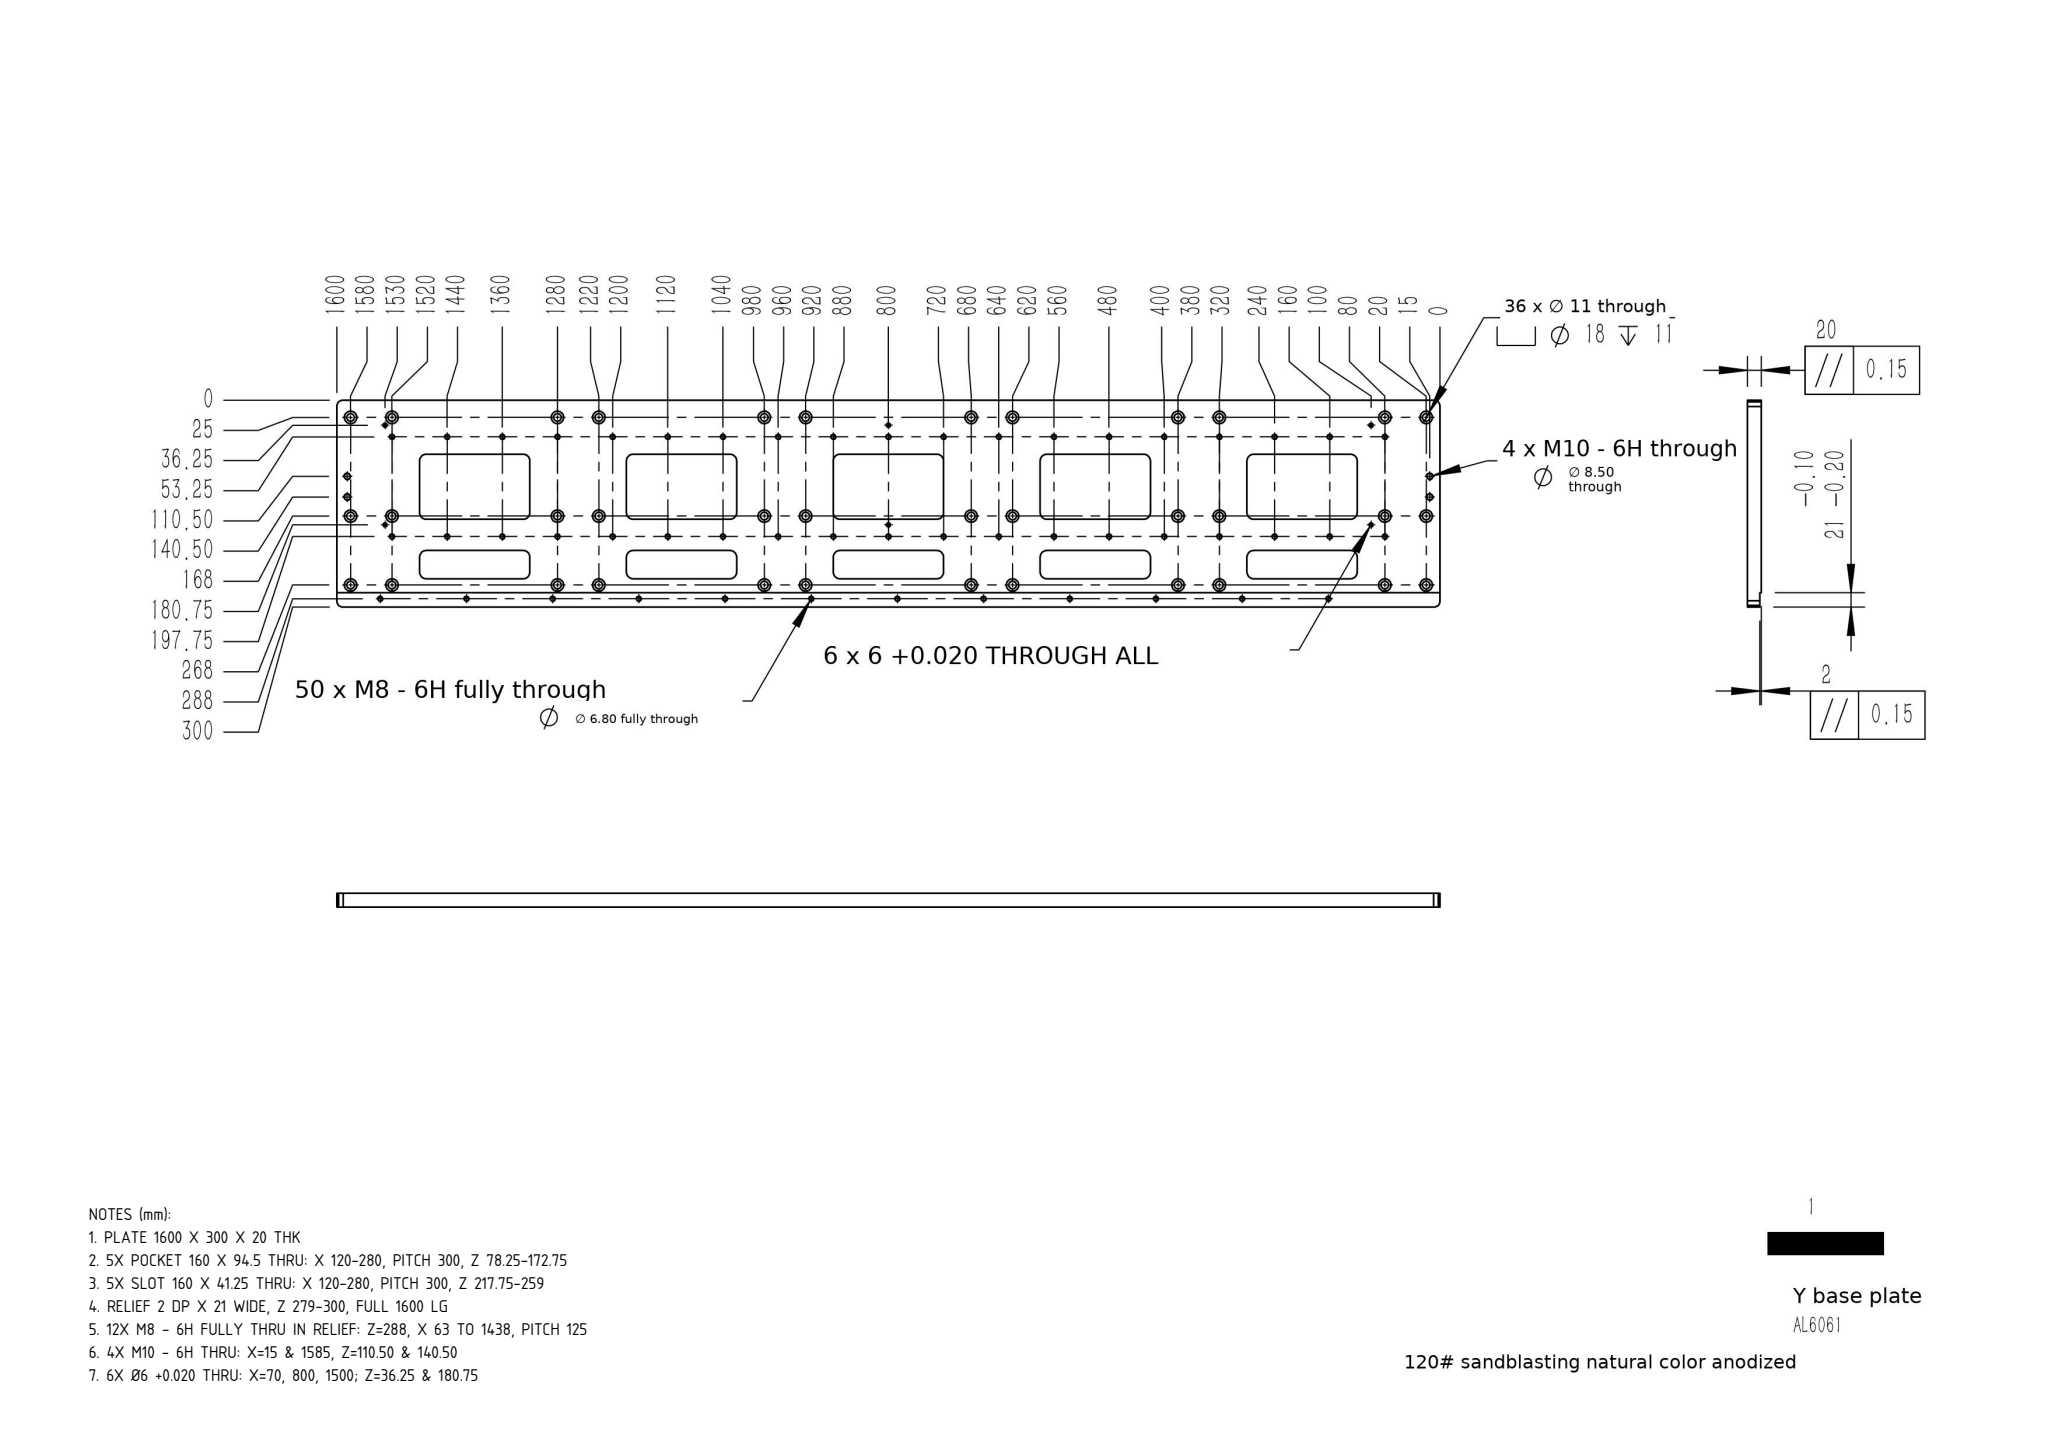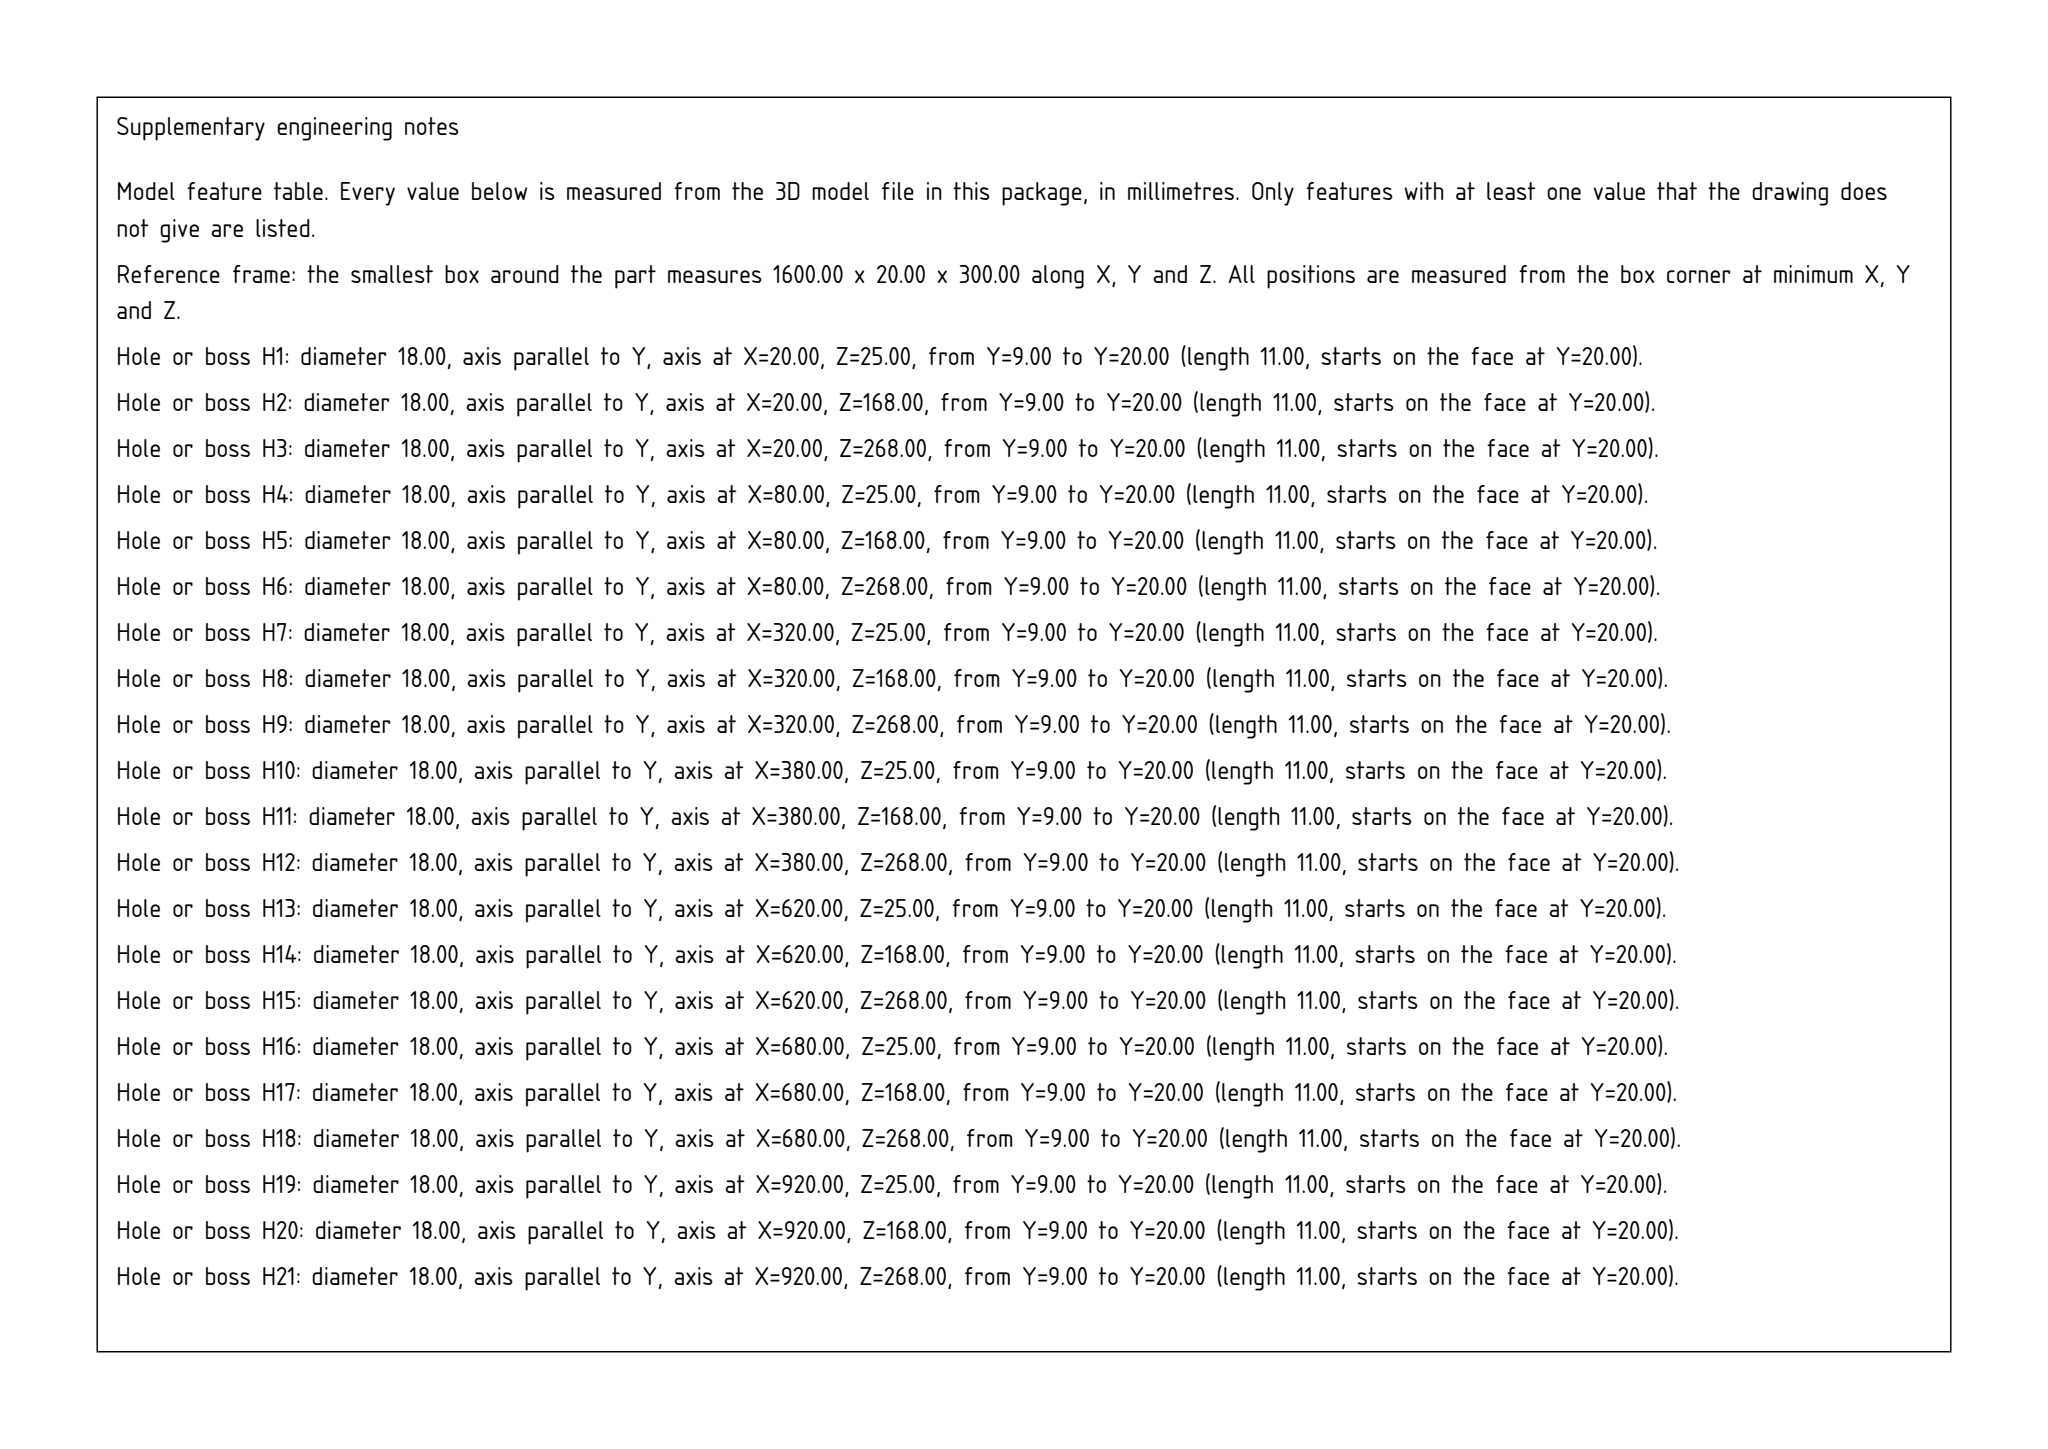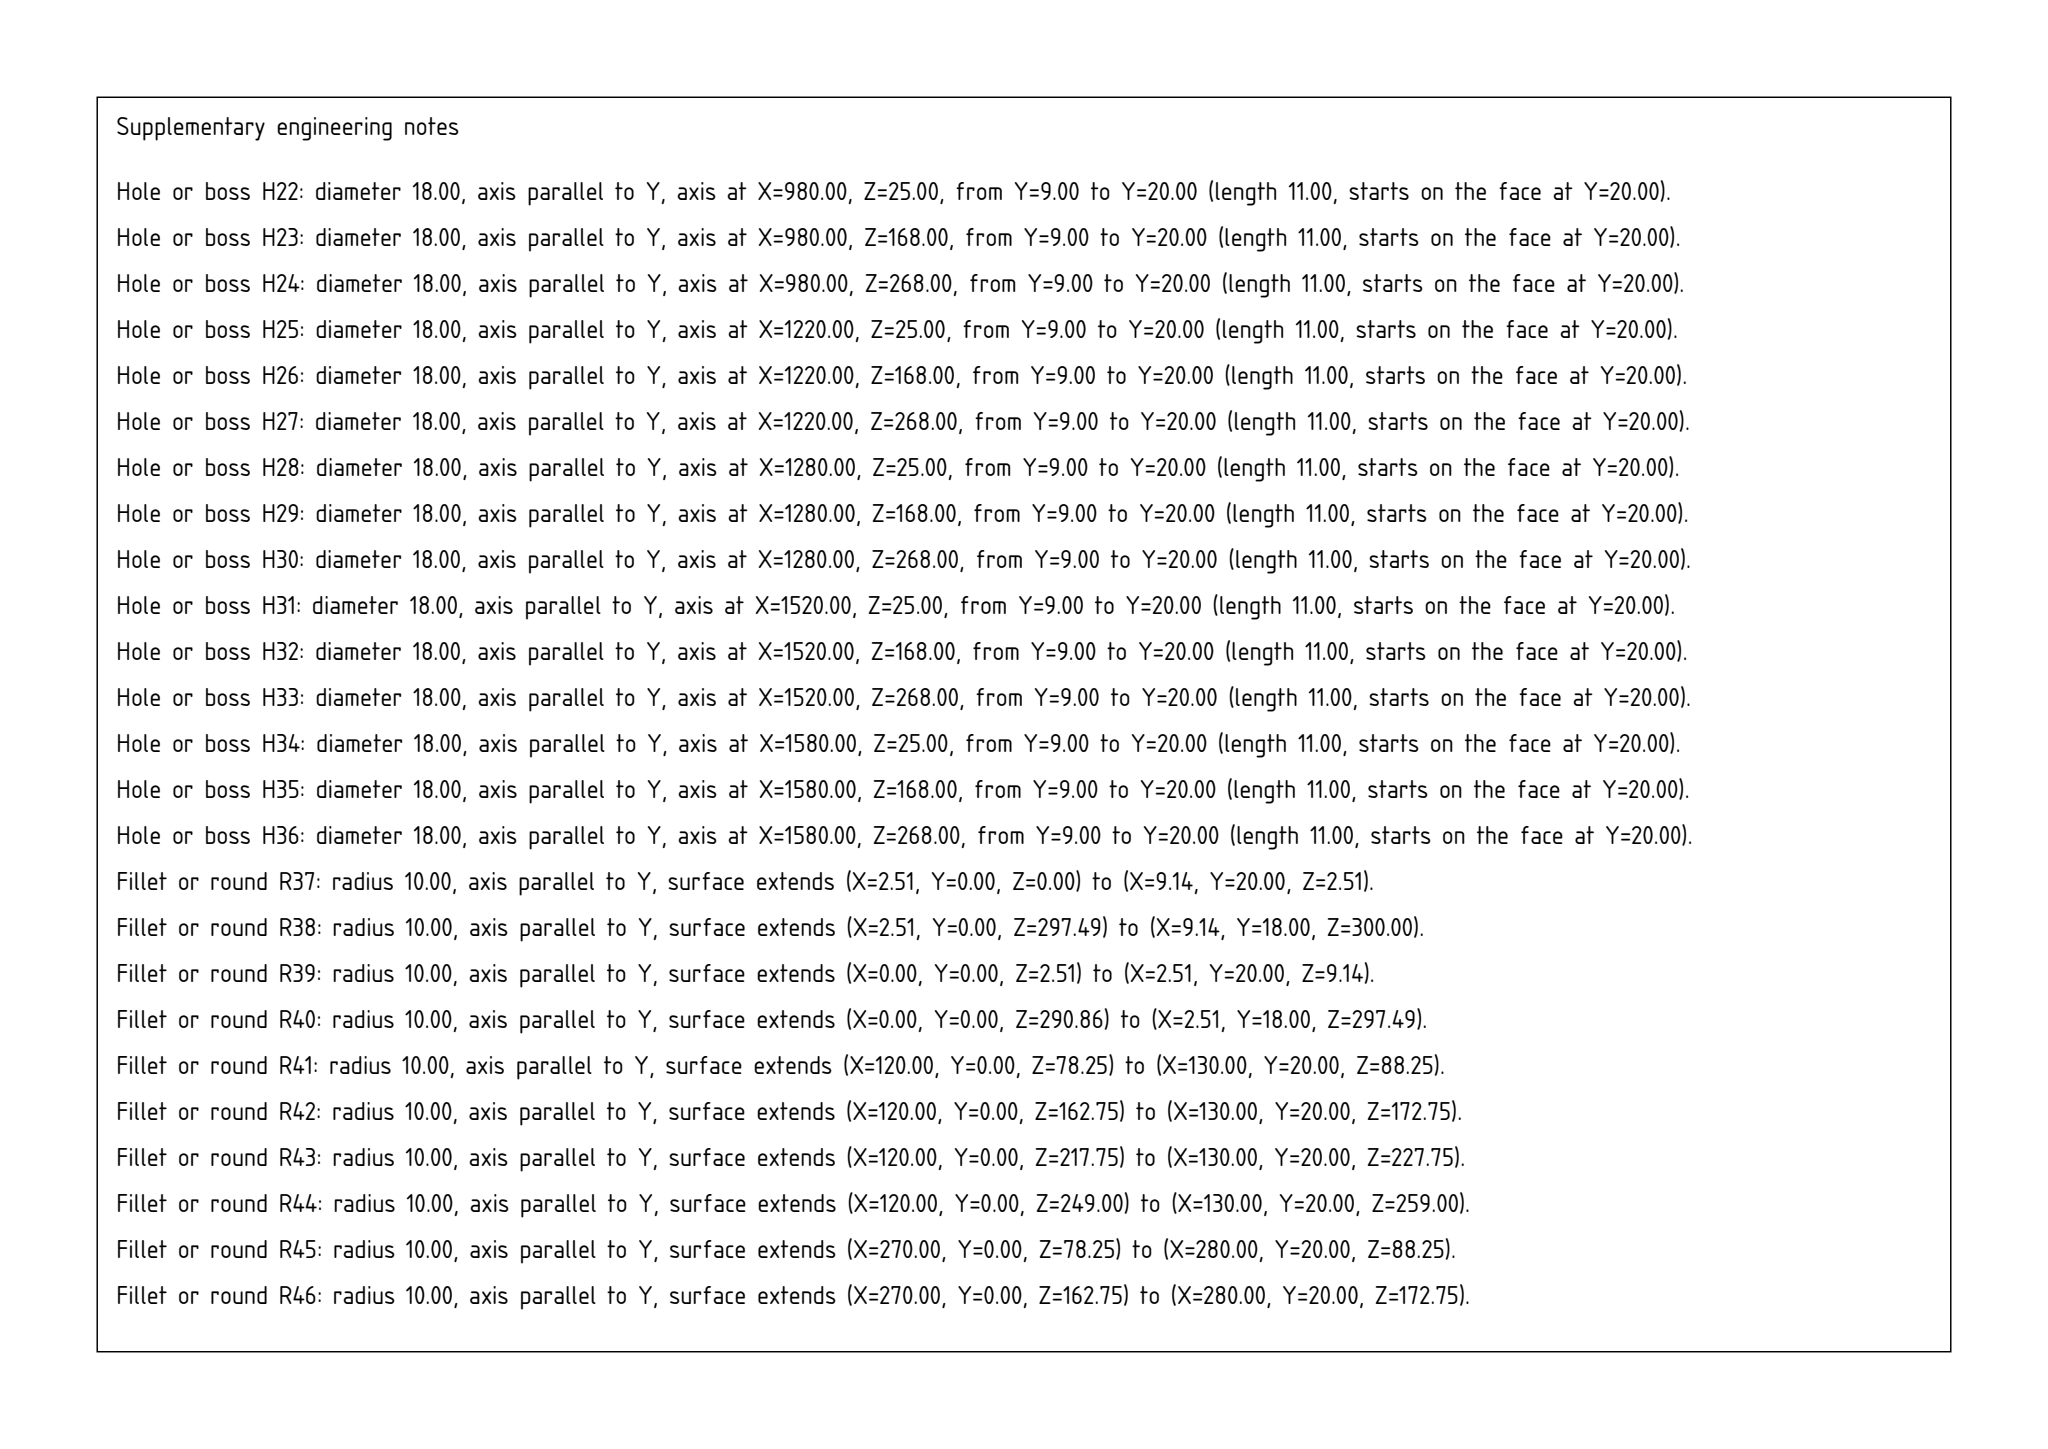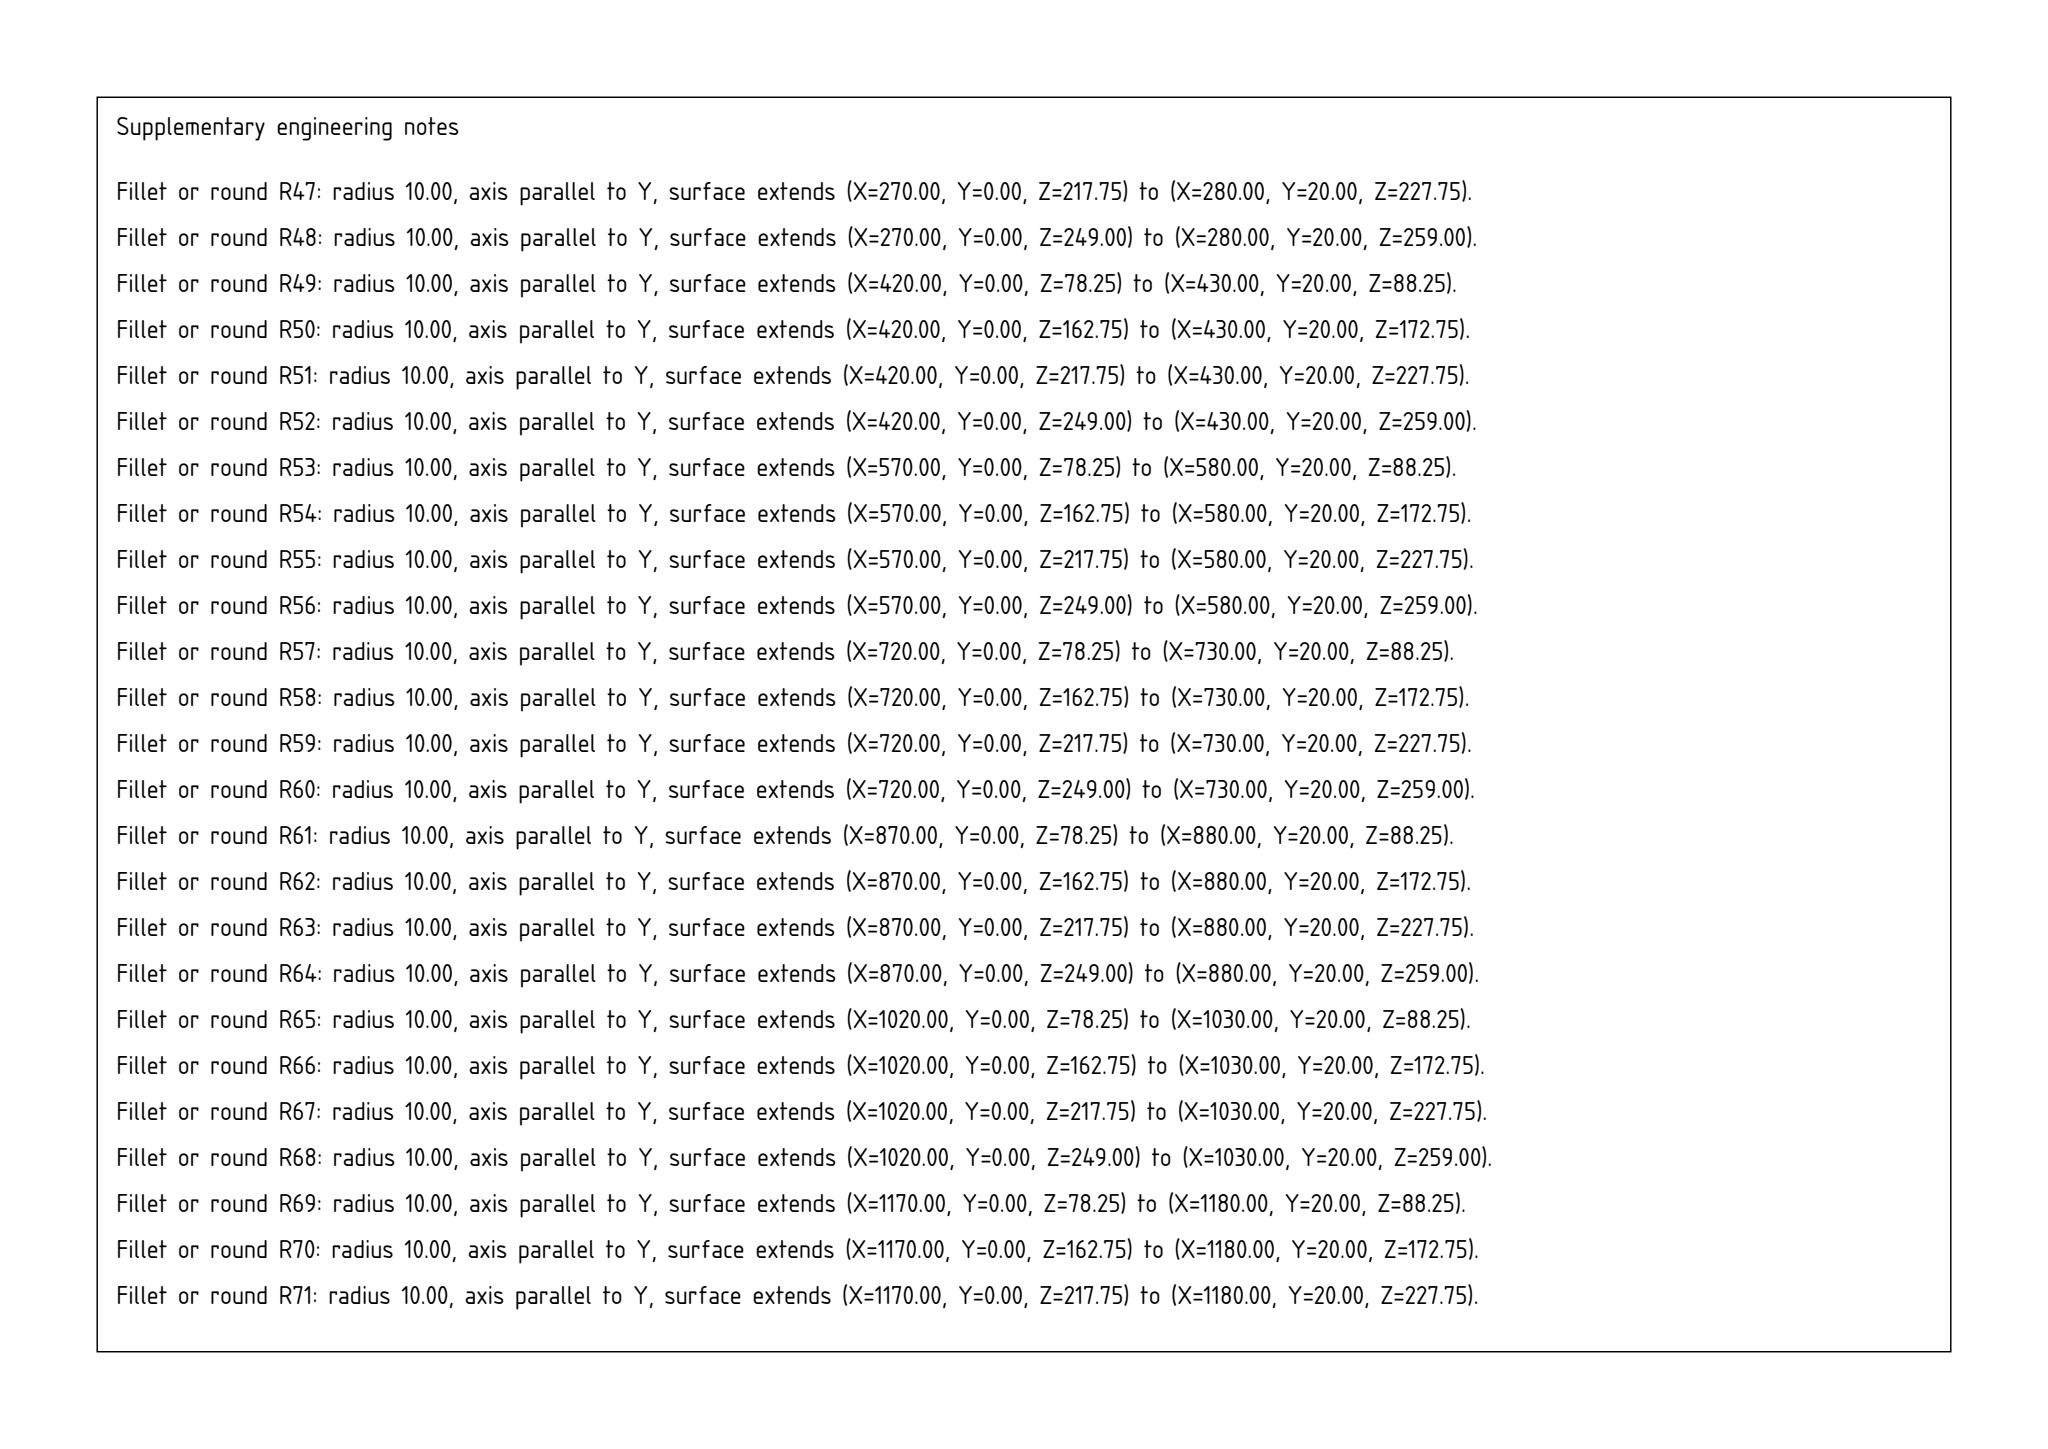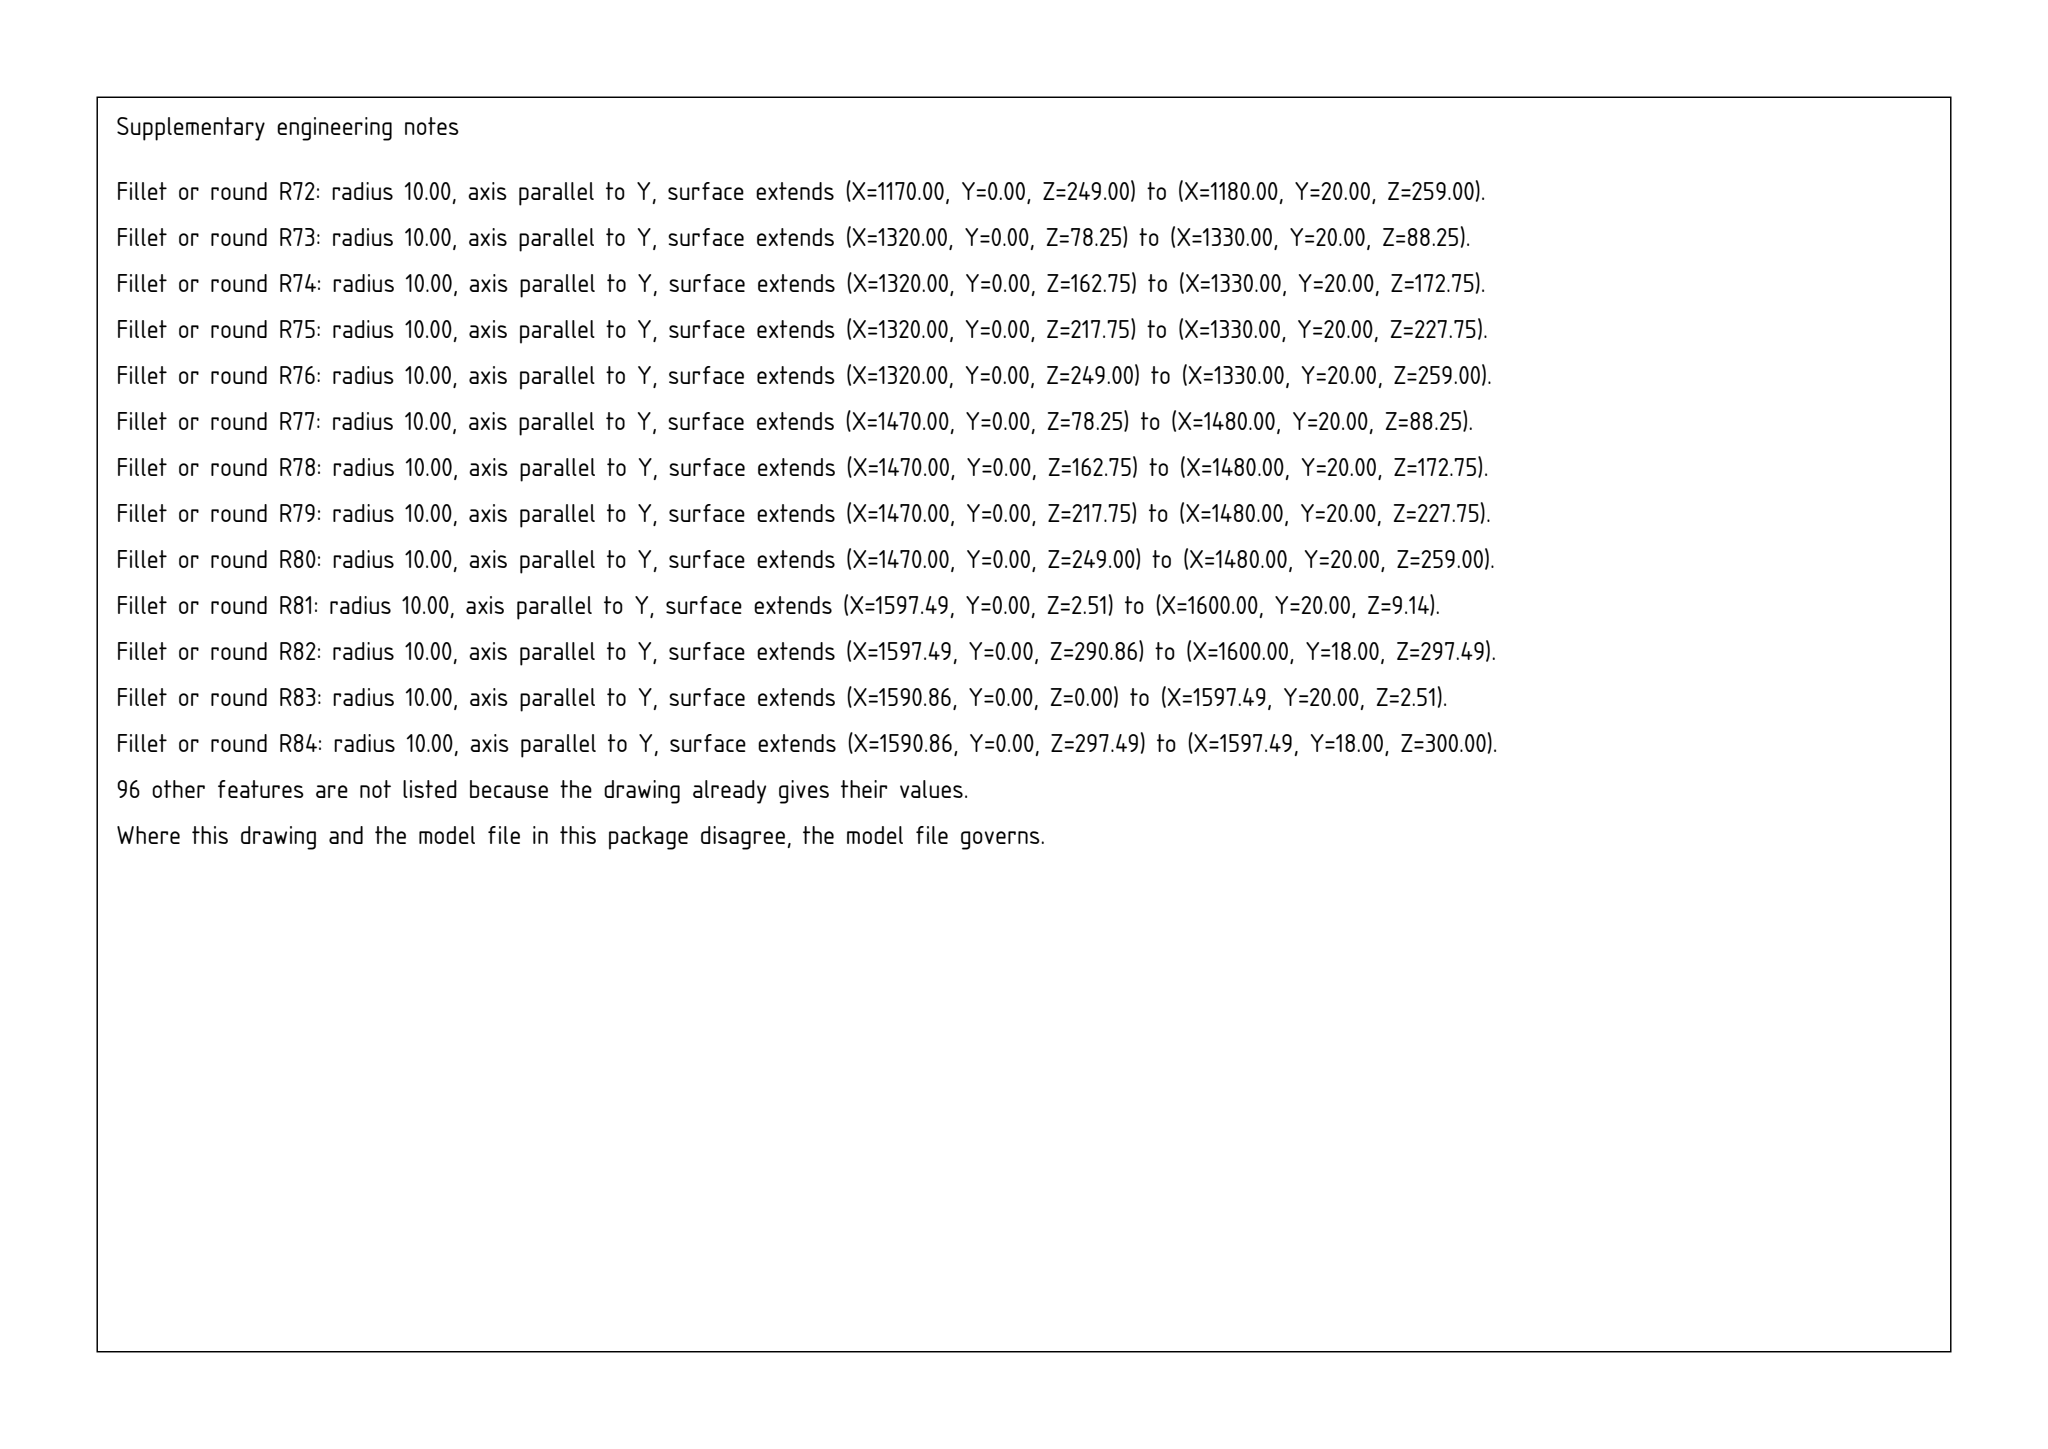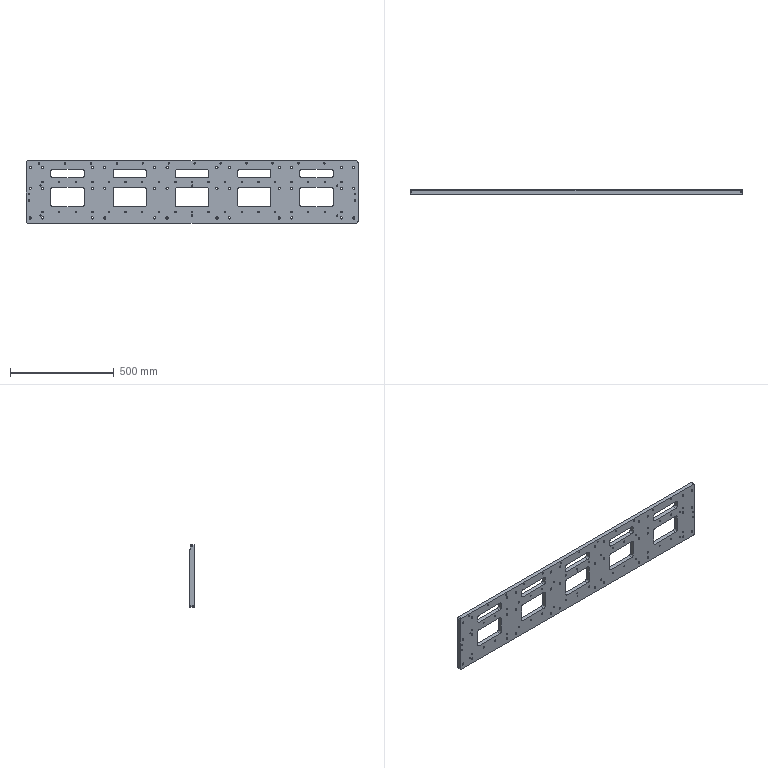Part | SolidWorks | mm | 1 solid | 396 faces | box 1600 x 20 x 300 mm | volume 7201753 mm3 | cylinder 312 | plane 84 | commonest cylinder face diameters 6.8 x100 18 x72 11 x72 20 x48 6 x12 8.5 x8
Drawing notes:
PLATE 1600 X 300 X 20 THK | from the solid: bbox_xyz 1600 x 300 x 20
5X POCKET 160 X 94.5 THRU: X 120-280, PITCH 300, Z 78.25-172.75 | from the solid: x planes 120/280,420/580,720/880,1020/1180,1320/1480; z 78.25 & 172.75 (5 each)
5X SLOT 160 X 41.25 THRU: X 120-280, PITCH 300, Z 217.75-259 | from the solid: same x plane pairs; z planes 217.75 & 259.0 (5 each)
RELIEF 2 DP X 21 WIDE, Z 279-300, FULL 1600 LG | from the solid: y plane 18 (1); z planes 279.0 & 300; 6.8 holes at z=288 len 18
12X M8 - 6H FULLY THRU IN RELIEF: Z=288, X 63 TO 1438, PITCH 125 | from the solid: Ø6.8 y-axis holes at z=288, x=63,188,...,1438, len 18
4X M10 - 6H THRU: X=15 & 1585, Z=110.50 & 140.50 | from the solid: Ø8.5 y-axis holes at x=15 and 1585, z=110.5 & 140.5
6X Ø6 +0.020 THRU: X=70, 800, 1500; Z=36.25 & 180.75 | from the solid: Ø6 cyl, axis y, len 20 at x=70,800,1500 x z=36.25,180.75